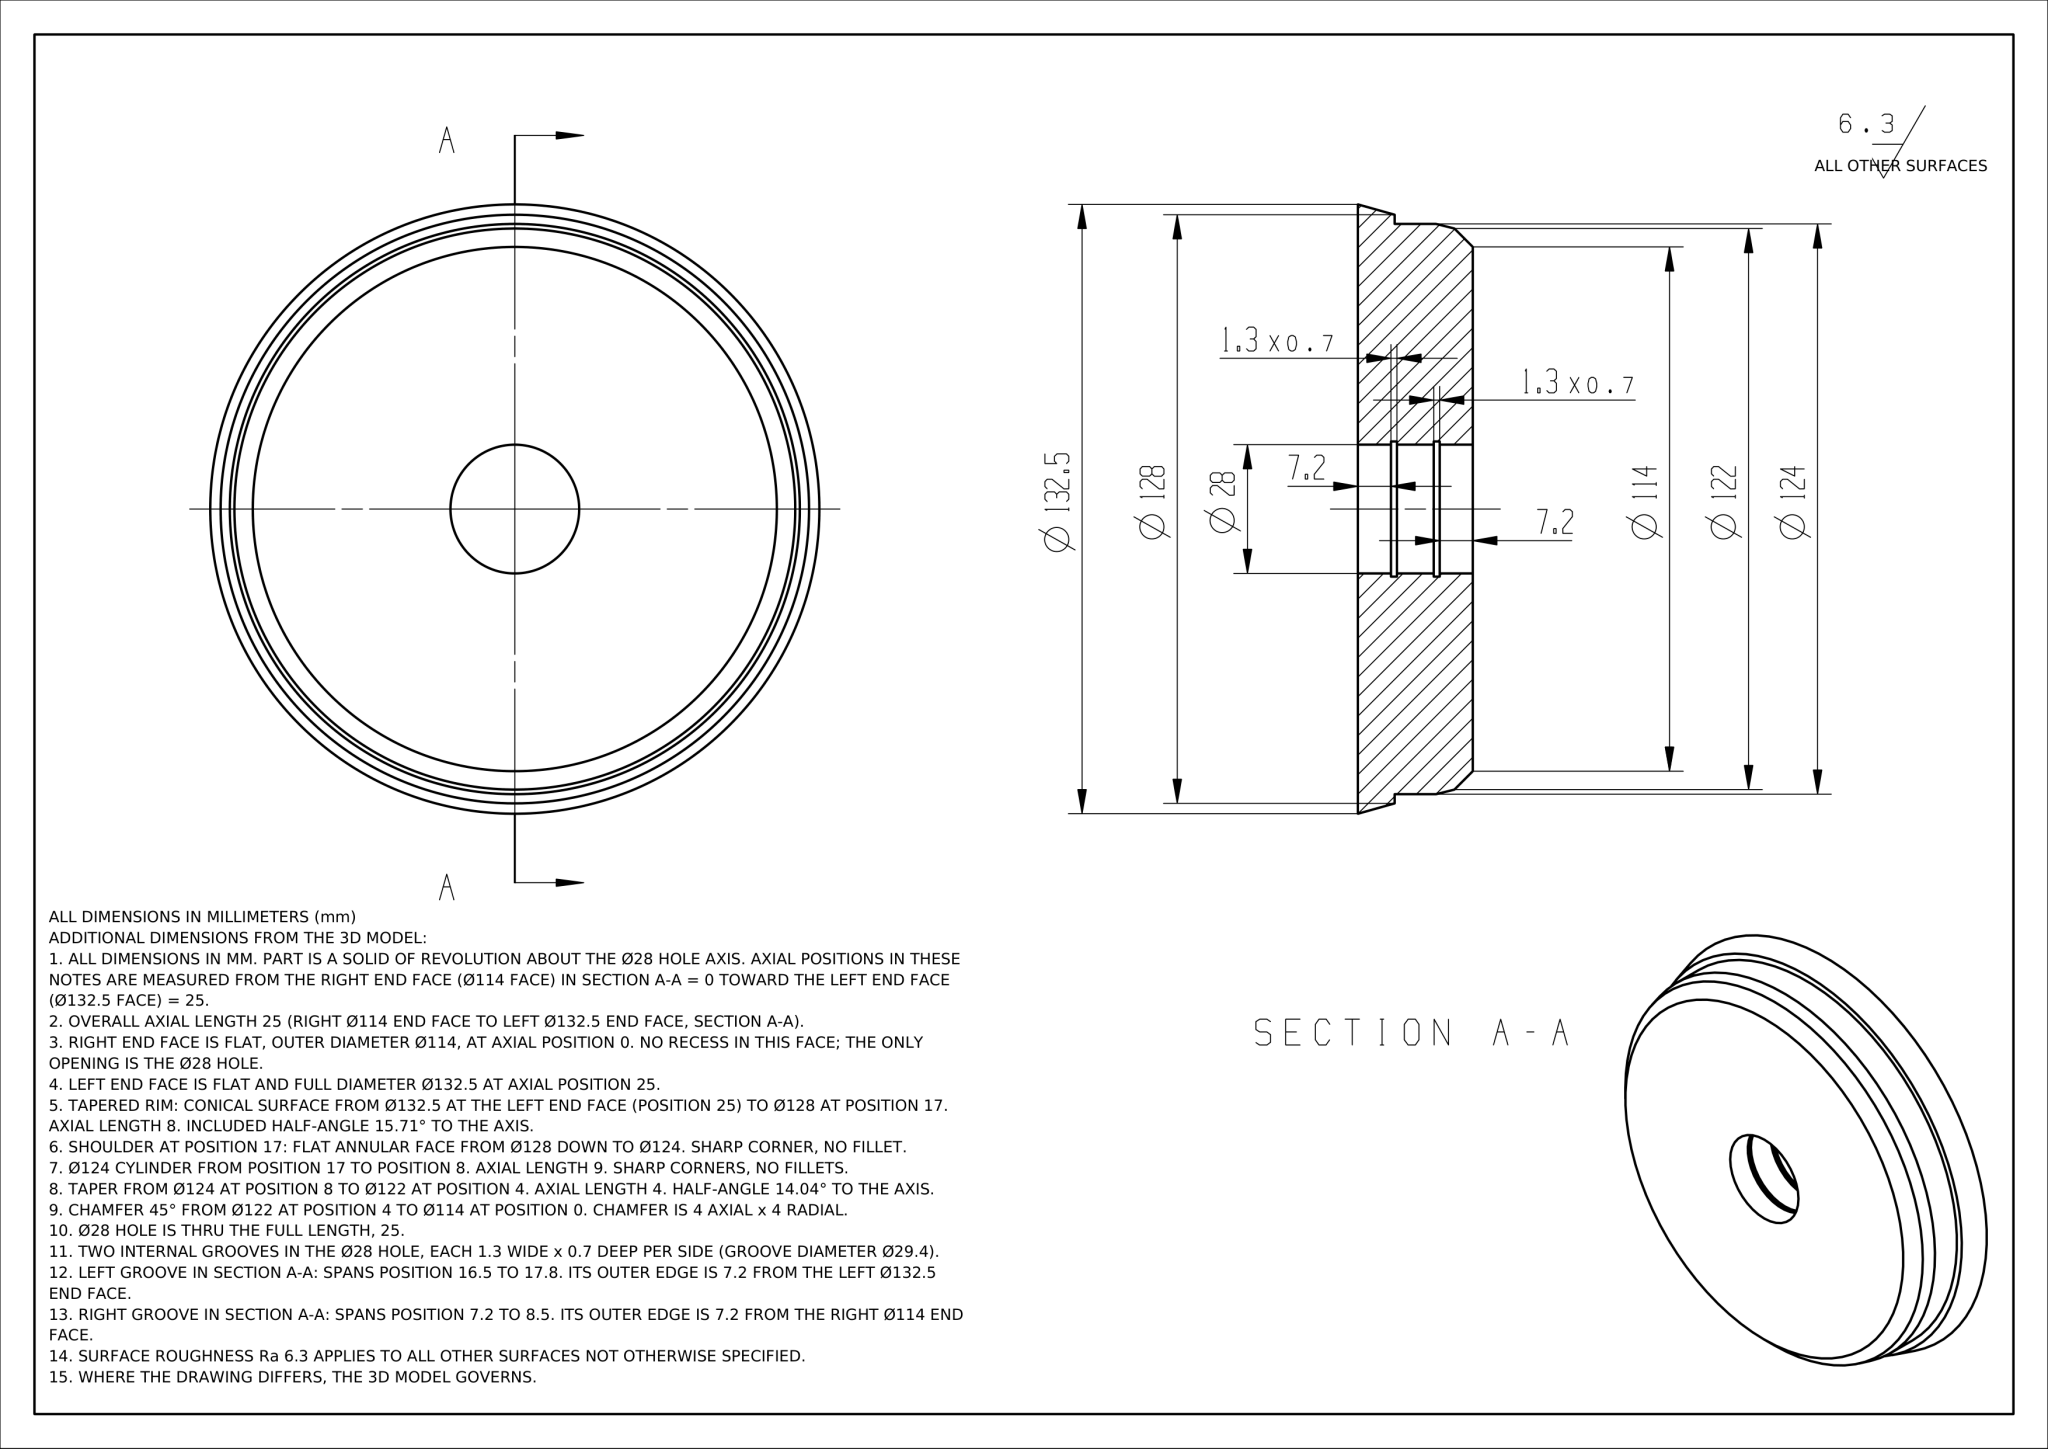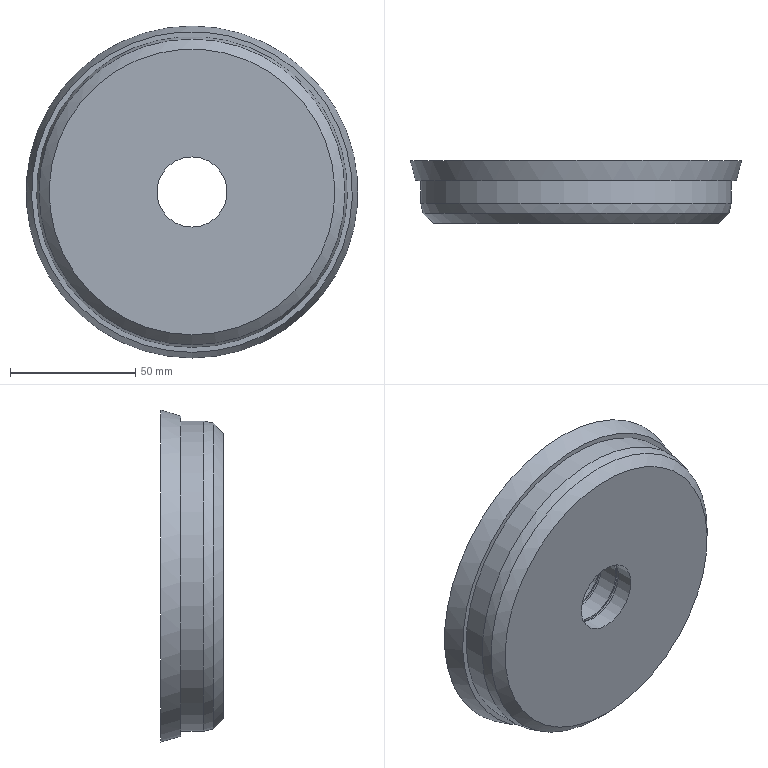Part | NX | mm | 1 solid | 16 faces | box 132.5 x 25 x 132.5 mm | volume 291024 mm3 | plane 7 | cylinder 6 | cone 3 | commonest cylinder face diameters 28 x3 29.4 x2 124 x1
STEP:
#1=CARTESIAN_POINT('',(0.,0.,0.));
#2=DIRECTION('',(0.,0.,1.));
#3=DIRECTION('',(1.,0.,0.));
#4=AXIS2_PLACEMENT_3D('',#1,#2,#3);
#5=(LENGTH_UNIT()NAMED_UNIT(*)SI_UNIT(.MILLI.,.METRE.));
#6=UNCERTAINTY_MEASURE_WITH_UNIT(LENGTH_MEASURE(0.00002),#5,'','');
#7=(NAMED_UNIT(*)PLANE_ANGLE_UNIT()SI_UNIT($,.RADIAN.));
#8=PLANE_ANGLE_MEASURE_WITH_UNIT(PLANE_ANGLE_MEASURE(0.01745),#7);
#9=DIMENSIONAL_EXPONENTS(0.,0.,0.,0.,0.,0.,0.);
#10=(CONVERSION_BASED_UNIT('',#8)NAMED_UNIT(#9)PLANE_ANGLE_UNIT());
#11=(NAMED_UNIT(*)SI_UNIT($,.STERADIAN.)SOLID_ANGLE_UNIT());
#12=(GEOMETRIC_REPRESENTATION_CONTEXT(3)GLOBAL_UNCERTAINTY_ASSIGNED_CONTEXT((#6))GLOBAL_UNIT_ASSIGNED_CONTEXT((#5,#10,#11))REPRESENTATION_CONTEXT('',''));
#13=SHAPE_REPRESENTATION('',(#4),#12);
#14=CARTESIAN_POINT('',(0.,25.,-14.));
#15=VERTEX_POINT('',#14);
#16=CARTESIAN_POINT('',(0.,25.,0.));
#17=DIRECTION('',(0.,-1.,0.));
#18=DIRECTION('',(0.,0.,-1.));
#19=AXIS2_PLACEMENT_3D('',#16,#17,#18);
#20=CIRCLE('',#19,14.);
#21=EDGE_CURVE('',#15,#15,#20,.T.);
#22=ORIENTED_EDGE('',*,*,#21,.F.);
#23=EDGE_LOOP('',(#22));
#24=FACE_BOUND('',#23,.T.);
#25=CARTESIAN_POINT('',(0.,17.8,-14.));
#26=VERTEX_POINT('',#25);
#27=CARTESIAN_POINT('',(0.,17.8,0.));
#28=DIRECTION('',(0.,1.,0.));
#29=DIRECTION('',(0.,0.,-1.));
#30=AXIS2_PLACEMENT_3D('',#27,#28,#29);
#31=CIRCLE('',#30,14.);
#32=EDGE_CURVE('',#26,#26,#31,.T.);
#33=ORIENTED_EDGE('',*,*,#32,.F.);
#34=EDGE_LOOP('',(#33));
#35=FACE_BOUND('',#34,.T.);
#36=CARTESIAN_POINT('',(0.,0.,0.));
#37=DIRECTION('',(0.,-1.,0.));
#38=DIRECTION('',(0.,0.,-1.));
#39=AXIS2_PLACEMENT_3D('',#36,#37,#38);
#40=CYLINDRICAL_SURFACE('',#39,14.);
#41=ADVANCED_FACE('',(#24,#35),#40,.F.);
#42=CARTESIAN_POINT('',(0.,0.,-14.));
#43=VERTEX_POINT('',#42);
#44=CARTESIAN_POINT('',(0.,0.,0.));
#45=DIRECTION('',(0.,-1.,0.));
#46=DIRECTION('',(0.,0.,-1.));
#47=AXIS2_PLACEMENT_3D('',#44,#45,#46);
#48=CIRCLE('',#47,14.);
#49=EDGE_CURVE('',#43,#43,#48,.T.);
#50=ORIENTED_EDGE('',*,*,#49,.T.);
#51=EDGE_LOOP('',(#50));
#52=FACE_BOUND('',#51,.T.);
#53=CARTESIAN_POINT('',(0.,7.2,14.));
#54=VERTEX_POINT('',#53);
#55=CARTESIAN_POINT('',(0.,7.2,0.));
#56=DIRECTION('',(0.,-1.,0.));
#57=DIRECTION('',(0.,0.,1.));
#58=AXIS2_PLACEMENT_3D('',#55,#56,#57);
#59=CIRCLE('',#58,14.);
#60=EDGE_CURVE('',#54,#54,#59,.T.);
#61=ORIENTED_EDGE('',*,*,#60,.F.);
#62=EDGE_LOOP('',(#61));
#63=FACE_BOUND('',#62,.T.);
#64=CARTESIAN_POINT('',(0.,0.,0.));
#65=DIRECTION('',(0.,-1.,0.));
#66=DIRECTION('',(0.,0.,-1.));
#67=AXIS2_PLACEMENT_3D('',#64,#65,#66);
#68=CYLINDRICAL_SURFACE('',#67,14.);
#69=ADVANCED_FACE('',(#52,#63),#68,.F.);
#70=ORIENTED_EDGE('',*,*,#49,.F.);
#71=EDGE_LOOP('',(#70));
#72=FACE_BOUND('',#71,.T.);
#73=CARTESIAN_POINT('',(0.,-0.,-57.));
#74=VERTEX_POINT('',#73);
#75=CARTESIAN_POINT('',(0.,-0.,0.));
#76=DIRECTION('',(0.,-1.,0.));
#77=DIRECTION('',(0.,0.,-1.));
#78=AXIS2_PLACEMENT_3D('',#75,#76,#77);
#79=CIRCLE('',#78,57.);
#80=EDGE_CURVE('',#74,#74,#79,.T.);
#81=ORIENTED_EDGE('',*,*,#80,.T.);
#82=EDGE_LOOP('',(#81));
#83=FACE_BOUND('',#82,.T.);
#84=CARTESIAN_POINT('',(0.,-0.,57.));
#85=DIRECTION('',(0.,1.,0.));
#86=DIRECTION('',(0.,0.,1.));
#87=AXIS2_PLACEMENT_3D('',#84,#85,#86);
#88=PLANE('',#87);
#89=ADVANCED_FACE('',(#72,#83),#88,.F.);
#90=CARTESIAN_POINT('',(0.,16.5,-14.));
#91=VERTEX_POINT('',#90);
#92=CARTESIAN_POINT('',(0.,16.5,0.));
#93=DIRECTION('',(0.,1.,0.));
#94=DIRECTION('',(0.,0.,-1.));
#95=AXIS2_PLACEMENT_3D('',#92,#93,#94);
#96=CIRCLE('',#95,14.);
#97=EDGE_CURVE('',#91,#91,#96,.T.);
#98=ORIENTED_EDGE('',*,*,#97,.T.);
#99=EDGE_LOOP('',(#98));
#100=FACE_BOUND('',#99,.T.);
#101=CARTESIAN_POINT('',(0.,8.5,14.));
#102=VERTEX_POINT('',#101);
#103=CARTESIAN_POINT('',(0.,8.5,0.));
#104=DIRECTION('',(0.,-1.,0.));
#105=DIRECTION('',(0.,0.,1.));
#106=AXIS2_PLACEMENT_3D('',#103,#104,#105);
#107=CIRCLE('',#106,14.);
#108=EDGE_CURVE('',#102,#102,#107,.T.);
#109=ORIENTED_EDGE('',*,*,#108,.T.);
#110=EDGE_LOOP('',(#109));
#111=FACE_BOUND('',#110,.T.);
#112=CARTESIAN_POINT('',(0.,0.,0.));
#113=DIRECTION('',(0.,-1.,0.));
#114=DIRECTION('',(0.,0.,-1.));
#115=AXIS2_PLACEMENT_3D('',#112,#113,#114);
#116=CYLINDRICAL_SURFACE('',#115,14.);
#117=ADVANCED_FACE('',(#100,#111),#116,.F.);
#118=CARTESIAN_POINT('',(0.,25.,-66.25));
#119=VERTEX_POINT('',#118);
#120=CARTESIAN_POINT('',(0.,25.,0.));
#121=DIRECTION('',(0.,-1.,0.));
#122=DIRECTION('',(0.,0.,-1.));
#123=AXIS2_PLACEMENT_3D('',#120,#121,#122);
#124=CIRCLE('',#123,66.25);
#125=EDGE_CURVE('',#119,#119,#124,.T.);
#126=ORIENTED_EDGE('',*,*,#125,.F.);
#127=EDGE_LOOP('',(#126));
#128=FACE_BOUND('',#127,.T.);
#129=ORIENTED_EDGE('',*,*,#21,.T.);
#130=EDGE_LOOP('',(#129));
#131=FACE_BOUND('',#130,.T.);
#132=CARTESIAN_POINT('',(0.,25.,14.));
#133=DIRECTION('',(0.,-1.,0.));
#134=DIRECTION('',(0.,0.,-1.));
#135=AXIS2_PLACEMENT_3D('',#132,#133,#134);
#136=PLANE('',#135);
#137=ADVANCED_FACE('',(#128,#131),#136,.F.);
#138=CARTESIAN_POINT('',(0.,17.,-64.));
#139=VERTEX_POINT('',#138);
#140=CARTESIAN_POINT('',(0.,17.,0.));
#141=DIRECTION('',(0.,-1.,0.));
#142=DIRECTION('',(0.,0.,-1.));
#143=AXIS2_PLACEMENT_3D('',#140,#141,#142);
#144=CIRCLE('',#143,64.);
#145=EDGE_CURVE('',#139,#139,#144,.T.);
#146=ORIENTED_EDGE('',*,*,#145,.F.);
#147=EDGE_LOOP('',(#146));
#148=FACE_BOUND('',#147,.T.);
#149=ORIENTED_EDGE('',*,*,#125,.T.);
#150=EDGE_LOOP('',(#149));
#151=FACE_BOUND('',#150,.T.);
#152=CARTESIAN_POINT('',(0.,25.,0.));
#153=DIRECTION('',(0.,1.,0.));
#154=DIRECTION('',(0.,-0.,1.));
#155=AXIS2_PLACEMENT_3D('',#152,#153,#154);
#156=CONICAL_SURFACE('',#155,66.25,15.709);
#157=ADVANCED_FACE('',(#148,#151),#156,.T.);
#158=CARTESIAN_POINT('',(0.,17.,-62.));
#159=VERTEX_POINT('',#158);
#160=CARTESIAN_POINT('',(0.,17.,0.));
#161=DIRECTION('',(0.,-1.,0.));
#162=DIRECTION('',(0.,0.,-1.));
#163=AXIS2_PLACEMENT_3D('',#160,#161,#162);
#164=CIRCLE('',#163,62.);
#165=EDGE_CURVE('',#159,#159,#164,.T.);
#166=ORIENTED_EDGE('',*,*,#165,.F.);
#167=EDGE_LOOP('',(#166));
#168=FACE_BOUND('',#167,.T.);
#169=ORIENTED_EDGE('',*,*,#145,.T.);
#170=EDGE_LOOP('',(#169));
#171=FACE_BOUND('',#170,.T.);
#172=CARTESIAN_POINT('',(0.,17.,64.));
#173=DIRECTION('',(0.,1.,0.));
#174=DIRECTION('',(0.,0.,1.));
#175=AXIS2_PLACEMENT_3D('',#172,#173,#174);
#176=PLANE('',#175);
#177=ADVANCED_FACE('',(#168,#171),#176,.F.);
#178=CARTESIAN_POINT('',(0.,8.,-62.));
#179=VERTEX_POINT('',#178);
#180=CARTESIAN_POINT('',(0.,8.,0.));
#181=DIRECTION('',(0.,-1.,0.));
#182=DIRECTION('',(0.,0.,-1.));
#183=AXIS2_PLACEMENT_3D('',#180,#181,#182);
#184=CIRCLE('',#183,62.);
#185=EDGE_CURVE('',#179,#179,#184,.T.);
#186=ORIENTED_EDGE('',*,*,#185,.F.);
#187=EDGE_LOOP('',(#186));
#188=FACE_BOUND('',#187,.T.);
#189=ORIENTED_EDGE('',*,*,#165,.T.);
#190=EDGE_LOOP('',(#189));
#191=FACE_BOUND('',#190,.T.);
#192=CARTESIAN_POINT('',(0.,0.,0.));
#193=DIRECTION('',(0.,-1.,0.));
#194=DIRECTION('',(0.,0.,-1.));
#195=AXIS2_PLACEMENT_3D('',#192,#193,#194);
#196=CYLINDRICAL_SURFACE('',#195,62.);
#197=ADVANCED_FACE('',(#188,#191),#196,.T.);
#198=CARTESIAN_POINT('',(0.,4.,-61.));
#199=VERTEX_POINT('',#198);
#200=CARTESIAN_POINT('',(0.,4.,0.));
#201=DIRECTION('',(0.,-1.,0.));
#202=DIRECTION('',(0.,0.,-1.));
#203=AXIS2_PLACEMENT_3D('',#200,#201,#202);
#204=CIRCLE('',#203,61.);
#205=EDGE_CURVE('',#199,#199,#204,.T.);
#206=ORIENTED_EDGE('',*,*,#205,.F.);
#207=EDGE_LOOP('',(#206));
#208=FACE_BOUND('',#207,.T.);
#209=ORIENTED_EDGE('',*,*,#185,.T.);
#210=EDGE_LOOP('',(#209));
#211=FACE_BOUND('',#210,.T.);
#212=CARTESIAN_POINT('',(0.,8.,0.));
#213=DIRECTION('',(0.,1.,0.));
#214=DIRECTION('',(0.,0.,1.));
#215=AXIS2_PLACEMENT_3D('',#212,#213,#214);
#216=CONICAL_SURFACE('',#215,62.,14.036);
#217=ADVANCED_FACE('',(#208,#211),#216,.T.);
#218=ORIENTED_EDGE('',*,*,#80,.F.);
#219=EDGE_LOOP('',(#218));
#220=FACE_BOUND('',#219,.T.);
#221=ORIENTED_EDGE('',*,*,#205,.T.);
#222=EDGE_LOOP('',(#221));
#223=FACE_BOUND('',#222,.T.);
#224=CARTESIAN_POINT('',(0.,4.,0.));
#225=DIRECTION('',(0.,1.,0.));
#226=DIRECTION('',(0.,0.,1.));
#227=AXIS2_PLACEMENT_3D('',#224,#225,#226);
#228=CONICAL_SURFACE('',#227,61.,45.);
#229=ADVANCED_FACE('',(#220,#223),#228,.T.);
#230=CARTESIAN_POINT('',(0.,7.2,14.7));
#231=VERTEX_POINT('',#230);
#232=CARTESIAN_POINT('',(0.,7.2,0.));
#233=DIRECTION('',(0.,-1.,0.));
#234=DIRECTION('',(0.,0.,1.));
#235=AXIS2_PLACEMENT_3D('',#232,#233,#234);
#236=CIRCLE('',#235,14.7);
#237=EDGE_CURVE('',#231,#231,#236,.T.);
#238=ORIENTED_EDGE('',*,*,#237,.F.);
#239=EDGE_LOOP('',(#238));
#240=FACE_BOUND('',#239,.T.);
#241=ORIENTED_EDGE('',*,*,#60,.T.);
#242=EDGE_LOOP('',(#241));
#243=FACE_BOUND('',#242,.T.);
#244=CARTESIAN_POINT('',(0.,7.2,0.));
#245=DIRECTION('',(0.,1.,0.));
#246=DIRECTION('',(0.,0.,1.));
#247=AXIS2_PLACEMENT_3D('',#244,#245,#246);
#248=PLANE('',#247);
#249=ADVANCED_FACE('',(#240,#243),#248,.T.);
#250=CARTESIAN_POINT('',(0.,8.5,14.7));
#251=VERTEX_POINT('',#250);
#252=CARTESIAN_POINT('',(0.,8.5,0.));
#253=DIRECTION('',(0.,-1.,0.));
#254=DIRECTION('',(0.,0.,1.));
#255=AXIS2_PLACEMENT_3D('',#252,#253,#254);
#256=CIRCLE('',#255,14.7);
#257=EDGE_CURVE('',#251,#251,#256,.T.);
#258=ORIENTED_EDGE('',*,*,#257,.T.);
#259=EDGE_LOOP('',(#258));
#260=FACE_BOUND('',#259,.T.);
#261=ORIENTED_EDGE('',*,*,#108,.F.);
#262=EDGE_LOOP('',(#261));
#263=FACE_BOUND('',#262,.T.);
#264=CARTESIAN_POINT('',(0.,8.5,0.));
#265=DIRECTION('',(0.,1.,0.));
#266=DIRECTION('',(0.,0.,1.));
#267=AXIS2_PLACEMENT_3D('',#264,#265,#266);
#268=PLANE('',#267);
#269=ADVANCED_FACE('',(#260,#263),#268,.F.);
#270=ORIENTED_EDGE('',*,*,#257,.F.);
#271=EDGE_LOOP('',(#270));
#272=FACE_BOUND('',#271,.T.);
#273=ORIENTED_EDGE('',*,*,#237,.T.);
#274=EDGE_LOOP('',(#273));
#275=FACE_BOUND('',#274,.T.);
#276=CARTESIAN_POINT('',(0.,7.35,0.));
#277=DIRECTION('',(0.,1.,0.));
#278=DIRECTION('',(0.,0.,1.));
#279=AXIS2_PLACEMENT_3D('',#276,#277,#278);
#280=CYLINDRICAL_SURFACE('',#279,14.7);
#281=ADVANCED_FACE('',(#272,#275),#280,.F.);
#282=CARTESIAN_POINT('',(0.,16.5,-14.7));
#283=VERTEX_POINT('',#282);
#284=CARTESIAN_POINT('',(0.,16.5,0.));
#285=DIRECTION('',(0.,-1.,0.));
#286=DIRECTION('',(0.,0.,-1.));
#287=AXIS2_PLACEMENT_3D('',#284,#285,#286);
#288=CIRCLE('',#287,14.7);
#289=EDGE_CURVE('',#283,#283,#288,.T.);
#290=ORIENTED_EDGE('',*,*,#289,.F.);
#291=EDGE_LOOP('',(#290));
#292=FACE_BOUND('',#291,.T.);
#293=ORIENTED_EDGE('',*,*,#97,.F.);
#294=EDGE_LOOP('',(#293));
#295=FACE_BOUND('',#294,.T.);
#296=CARTESIAN_POINT('',(0.,16.5,0.));
#297=DIRECTION('',(0.,-1.,0.));
#298=DIRECTION('',(0.,0.,-1.));
#299=AXIS2_PLACEMENT_3D('',#296,#297,#298);
#300=PLANE('',#299);
#301=ADVANCED_FACE('',(#292,#295),#300,.F.);
#302=CARTESIAN_POINT('',(0.,17.8,-14.7));
#303=VERTEX_POINT('',#302);
#304=CARTESIAN_POINT('',(0.,17.8,0.));
#305=DIRECTION('',(0.,-1.,0.));
#306=DIRECTION('',(0.,0.,-1.));
#307=AXIS2_PLACEMENT_3D('',#304,#305,#306);
#308=CIRCLE('',#307,14.7);
#309=EDGE_CURVE('',#303,#303,#308,.T.);
#310=ORIENTED_EDGE('',*,*,#309,.T.);
#311=EDGE_LOOP('',(#310));
#312=FACE_BOUND('',#311,.T.);
#313=ORIENTED_EDGE('',*,*,#32,.T.);
#314=EDGE_LOOP('',(#313));
#315=FACE_BOUND('',#314,.T.);
#316=CARTESIAN_POINT('',(0.,17.8,0.));
#317=DIRECTION('',(0.,-1.,0.));
#318=DIRECTION('',(0.,0.,-1.));
#319=AXIS2_PLACEMENT_3D('',#316,#317,#318);
#320=PLANE('',#319);
#321=ADVANCED_FACE('',(#312,#315),#320,.T.);
#322=ORIENTED_EDGE('',*,*,#289,.T.);
#323=EDGE_LOOP('',(#322));
#324=FACE_BOUND('',#323,.T.);
#325=ORIENTED_EDGE('',*,*,#309,.F.);
#326=EDGE_LOOP('',(#325));
#327=FACE_BOUND('',#326,.T.);
#328=CARTESIAN_POINT('',(0.,17.65,0.));
#329=DIRECTION('',(0.,-1.,0.));
#330=DIRECTION('',(0.,0.,-1.));
#331=AXIS2_PLACEMENT_3D('',#328,#329,#330);
#332=CYLINDRICAL_SURFACE('',#331,14.7);
#333=ADVANCED_FACE('',(#324,#327),#332,.F.);
#334=CLOSED_SHELL('',(#41,#69,#89,#117,#137,#157,#177,#197,#217,#229,#249,#269,#281,#301,#321,#333));
#335=MANIFOLD_SOLID_BREP('',#334);
#336=ADVANCED_BREP_SHAPE_REPRESENTATION('',(#335),#12);
#337=SHAPE_REPRESENTATION_RELATIONSHIP('','',#13,#336);
#338=PRESENTATION_LAYER_ASSIGNMENT('','',(#335));
#339=COLOUR_RGB('',0.4,0.4,0.4);
#340=FILL_AREA_STYLE_COLOUR('',#339);
#341=FILL_AREA_STYLE('',(#340));
#342=SURFACE_STYLE_FILL_AREA(#341);
#343=SURFACE_SIDE_STYLE('',(#342));
#344=SURFACE_STYLE_USAGE(.BOTH.,#343);
#345=PRESENTATION_STYLE_ASSIGNMENT((#344));
#346=STYLED_ITEM('',(#345),#335);
#347=MECHANICAL_DESIGN_GEOMETRIC_PRESENTATION_REPRESENTATION('',(#346),#12);